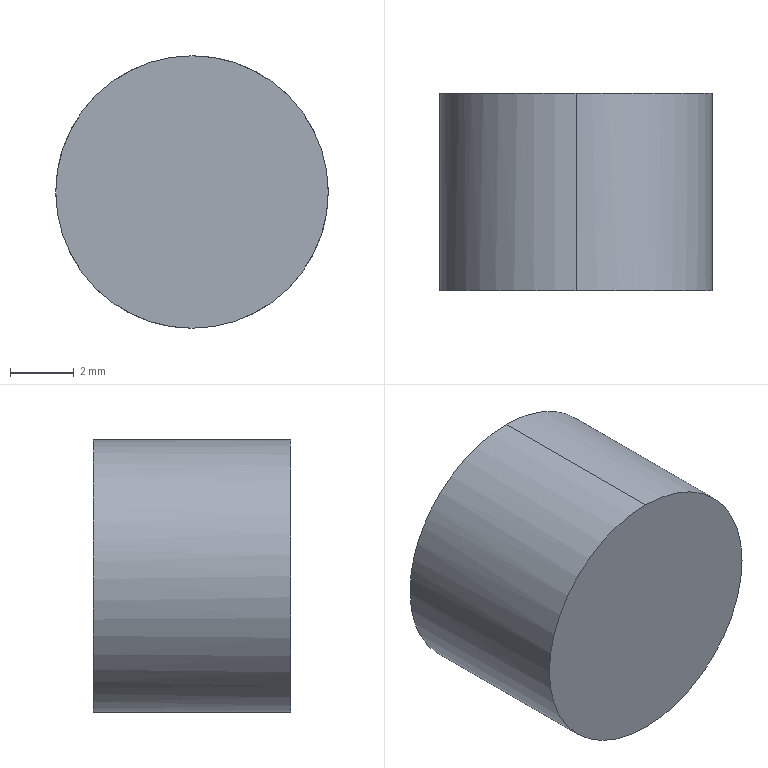Component | SolidWorks | MGPM20-20Z-M9P-1_MGP_Z_PLUG_20_9-1 | 1 solid | 11 faces | box 8.57 x 6.2 x 8.57 mm | volume 322 mm3 | plane 9 | cylinder 2 | commonest cylinder face diameters 8.566 x2
STEP:
#1=COLOUR_RGB('',0.7922,0.8196,0.9333);
#2=FILL_AREA_STYLE_COLOUR('',#1);
#3=FILL_AREA_STYLE('',(#2));
#4=SURFACE_STYLE_FILL_AREA(#3);
#5=SURFACE_SIDE_STYLE('',(#4));
#6=SURFACE_STYLE_USAGE(.BOTH.,#5);
#7=PRESENTATION_STYLE_ASSIGNMENT((#6));
#8=CARTESIAN_POINT('',(3.737,3.748,2.864));
#9=VERTEX_POINT('',#8);
#10=CARTESIAN_POINT('',(3.737,3.748,2.527));
#11=VERTEX_POINT('',#10);
#12=CARTESIAN_POINT('',(3.737,3.748,2.864));
#13=CARTESIAN_POINT('',(3.715,3.748,2.864));
#14=CARTESIAN_POINT('',(3.693,3.748,2.86));
#15=CARTESIAN_POINT('',(3.652,3.748,2.843));
#16=CARTESIAN_POINT('',(3.633,3.748,2.831));
#17=CARTESIAN_POINT('',(3.602,3.748,2.799));
#18=CARTESIAN_POINT('',(3.59,3.748,2.781));
#19=CARTESIAN_POINT('',(3.573,3.748,2.74));
#20=CARTESIAN_POINT('',(3.568,3.748,2.718));
#21=CARTESIAN_POINT('',(3.568,3.748,2.674));
#22=CARTESIAN_POINT('',(3.573,3.748,2.652));
#23=CARTESIAN_POINT('',(3.59,3.748,2.611));
#24=CARTESIAN_POINT('',(3.602,3.748,2.592));
#25=CARTESIAN_POINT('',(3.633,3.748,2.561));
#26=CARTESIAN_POINT('',(3.652,3.748,2.548));
#27=CARTESIAN_POINT('',(3.693,3.748,2.532));
#28=CARTESIAN_POINT('',(3.715,3.748,2.527));
#29=CARTESIAN_POINT('',(3.737,3.748,2.527));
#30=B_SPLINE_CURVE_WITH_KNOTS('',3,(#12,#13,#14,#15,#16,#17,#18,#19,#20,#21,#22,#23,#24,#25,#26,#27,#28,#29),.UNSPECIFIED.,.F.,.F.,(4,2,2,2,2,2,2,2,4),(0.,0.0625,0.125,0.1875,0.25,0.3125,0.375,0.4375,0.5),.UNSPECIFIED.);
#31=EDGE_CURVE('',#9,#11,#30,.T.);
#32=ORIENTED_EDGE('',*,*,#31,.T.);
#33=CARTESIAN_POINT('',(3.737,3.503,2.527));
#34=VERTEX_POINT('',#33);
#35=CARTESIAN_POINT('',(3.737,3.748,2.527));
#36=DIRECTION('',(0.,-1.,0.));
#37=VECTOR('',#36,39.37);
#38=LINE('',#35,#37);
#39=EDGE_CURVE('',#11,#34,#38,.T.);
#40=ORIENTED_EDGE('',*,*,#39,.T.);
#41=CARTESIAN_POINT('',(3.737,3.503,2.864));
#42=VERTEX_POINT('',#41);
#43=CARTESIAN_POINT('',(3.737,3.503,2.696));
#44=DIRECTION('',(0.,-1.,0.));
#45=DIRECTION('',(0.,0.,1.));
#46=AXIS2_PLACEMENT_3D('',#43,#44,#45);
#47=CIRCLE('',#46,0.1686);
#48=EDGE_CURVE('',#42,#34,#47,.T.);
#49=ORIENTED_EDGE('',*,*,#48,.F.);
#50=CARTESIAN_POINT('',(3.737,3.748,2.864));
#51=DIRECTION('',(0.,-1.,0.));
#52=VECTOR('',#51,39.37);
#53=LINE('',#50,#52);
#54=EDGE_CURVE('',#9,#42,#53,.T.);
#55=ORIENTED_EDGE('',*,*,#54,.F.);
#56=EDGE_LOOP('',(#32,#40,#49,#55));
#57=FACE_OUTER_BOUND('',#56,.T.);
#58=CARTESIAN_POINT('',(3.737,3.748,2.696));
#59=DIRECTION('',(0.,-1.,0.));
#60=DIRECTION('',(0.,0.,1.));
#61=AXIS2_PLACEMENT_3D('',#58,#59,#60);
#62=CYLINDRICAL_SURFACE('',#61,0.1686);
#63=ADVANCED_FACE('',(#57),#62,.T.);
#64=ORIENTED_EDGE('',*,*,#31,.F.);
#65=CARTESIAN_POINT('',(3.737,3.748,2.527));
#66=CARTESIAN_POINT('',(3.759,3.748,2.527));
#67=CARTESIAN_POINT('',(3.781,3.748,2.532));
#68=CARTESIAN_POINT('',(3.822,3.748,2.548));
#69=CARTESIAN_POINT('',(3.841,3.748,2.561));
#70=CARTESIAN_POINT('',(3.872,3.748,2.592));
#71=CARTESIAN_POINT('',(3.884,3.748,2.611));
#72=CARTESIAN_POINT('',(3.901,3.748,2.652));
#73=CARTESIAN_POINT('',(3.906,3.748,2.674));
#74=CARTESIAN_POINT('',(3.906,3.748,2.718));
#75=CARTESIAN_POINT('',(3.901,3.748,2.74));
#76=CARTESIAN_POINT('',(3.884,3.748,2.781));
#77=CARTESIAN_POINT('',(3.872,3.748,2.799));
#78=CARTESIAN_POINT('',(3.841,3.748,2.831));
#79=CARTESIAN_POINT('',(3.822,3.748,2.843));
#80=CARTESIAN_POINT('',(3.781,3.748,2.86));
#81=CARTESIAN_POINT('',(3.759,3.748,2.864));
#82=CARTESIAN_POINT('',(3.737,3.748,2.864));
#83=B_SPLINE_CURVE_WITH_KNOTS('',3,(#65,#66,#67,#68,#69,#70,#71,#72,#73,#74,#75,#76,#77,#78,#79,#80,#81,#82),.UNSPECIFIED.,.F.,.F.,(4,2,2,2,2,2,2,2,4),(0.5,0.5625,0.625,0.6875,0.75,0.8125,0.875,0.9375,1.),.UNSPECIFIED.);
#84=EDGE_CURVE('',#11,#9,#83,.T.);
#85=ORIENTED_EDGE('',*,*,#84,.F.);
#86=EDGE_LOOP('',(#64,#85));
#87=FACE_OUTER_BOUND('',#86,.T.);
#88=CARTESIAN_POINT('',(3.686,3.748,2.607));
#89=VERTEX_POINT('',#88);
#90=CARTESIAN_POINT('',(3.788,3.748,2.607));
#91=VERTEX_POINT('',#90);
#92=CARTESIAN_POINT('',(3.686,3.748,2.607));
#93=DIRECTION('',(1.,0.,-0.));
#94=VECTOR('',#93,39.37);
#95=LINE('',#92,#94);
#96=EDGE_CURVE('',#89,#91,#95,.T.);
#97=ORIENTED_EDGE('',*,*,#96,.T.);
#98=CARTESIAN_POINT('',(3.839,3.748,2.696));
#99=VERTEX_POINT('',#98);
#100=CARTESIAN_POINT('',(3.788,3.748,2.607));
#101=DIRECTION('',(0.5,0.,0.866));
#102=VECTOR('',#101,39.37);
#103=LINE('',#100,#102);
#104=EDGE_CURVE('',#91,#99,#103,.T.);
#105=ORIENTED_EDGE('',*,*,#104,.T.);
#106=CARTESIAN_POINT('',(3.788,3.748,2.784));
#107=VERTEX_POINT('',#106);
#108=CARTESIAN_POINT('',(3.839,3.748,2.696));
#109=DIRECTION('',(-0.5,0.,0.866));
#110=VECTOR('',#109,39.37);
#111=LINE('',#108,#110);
#112=EDGE_CURVE('',#99,#107,#111,.T.);
#113=ORIENTED_EDGE('',*,*,#112,.T.);
#114=CARTESIAN_POINT('',(3.686,3.748,2.784));
#115=VERTEX_POINT('',#114);
#116=CARTESIAN_POINT('',(3.788,3.748,2.784));
#117=DIRECTION('',(-1.,-0.,0.));
#118=VECTOR('',#117,39.37);
#119=LINE('',#116,#118);
#120=EDGE_CURVE('',#107,#115,#119,.T.);
#121=ORIENTED_EDGE('',*,*,#120,.T.);
#122=CARTESIAN_POINT('',(3.635,3.748,2.696));
#123=VERTEX_POINT('',#122);
#124=CARTESIAN_POINT('',(3.686,3.748,2.784));
#125=DIRECTION('',(-0.5,-0.,-0.866));
#126=VECTOR('',#125,39.37);
#127=LINE('',#124,#126);
#128=EDGE_CURVE('',#115,#123,#127,.T.);
#129=ORIENTED_EDGE('',*,*,#128,.T.);
#130=CARTESIAN_POINT('',(3.635,3.748,2.696));
#131=DIRECTION('',(0.5,-0.,-0.866));
#132=VECTOR('',#131,39.37);
#133=LINE('',#130,#132);
#134=EDGE_CURVE('',#123,#89,#133,.T.);
#135=ORIENTED_EDGE('',*,*,#134,.T.);
#136=EDGE_LOOP('',(#97,#105,#113,#121,#129,#135));
#137=FACE_BOUND('',#136,.T.);
#138=CARTESIAN_POINT('',(3.737,3.748,2.696));
#139=DIRECTION('',(0.,-1.,0.));
#140=DIRECTION('',(0.,0.,1.));
#141=AXIS2_PLACEMENT_3D('',#138,#139,#140);
#142=PLANE('',#141);
#143=ADVANCED_FACE('',(#87,#137),#142,.F.);
#144=ORIENTED_EDGE('',*,*,#134,.F.);
#145=CARTESIAN_POINT('',(3.635,3.669,2.696));
#146=VERTEX_POINT('',#145);
#147=CARTESIAN_POINT('',(3.635,3.669,2.696));
#148=DIRECTION('',(-0.,1.,-0.));
#149=VECTOR('',#148,39.37);
#150=LINE('',#147,#149);
#151=EDGE_CURVE('',#146,#123,#150,.T.);
#152=ORIENTED_EDGE('',*,*,#151,.F.);
#153=CARTESIAN_POINT('',(3.686,3.669,2.607));
#154=VERTEX_POINT('',#153);
#155=CARTESIAN_POINT('',(3.635,3.669,2.696));
#156=DIRECTION('',(0.5,-0.,-0.866));
#157=VECTOR('',#156,39.37);
#158=LINE('',#155,#157);
#159=EDGE_CURVE('',#146,#154,#158,.T.);
#160=ORIENTED_EDGE('',*,*,#159,.T.);
#161=CARTESIAN_POINT('',(3.686,3.669,2.607));
#162=DIRECTION('',(-0.,1.,-0.));
#163=VECTOR('',#162,39.37);
#164=LINE('',#161,#163);
#165=EDGE_CURVE('',#154,#89,#164,.T.);
#166=ORIENTED_EDGE('',*,*,#165,.T.);
#167=EDGE_LOOP('',(#144,#152,#160,#166));
#168=FACE_OUTER_BOUND('',#167,.T.);
#169=CARTESIAN_POINT('',(3.635,3.669,2.696));
#170=DIRECTION('',(0.866,0.,0.5));
#171=DIRECTION('',(-0.5,0.,0.866));
#172=AXIS2_PLACEMENT_3D('',#169,#170,#171);
#173=PLANE('',#172);
#174=ADVANCED_FACE('',(#168),#173,.T.);
#175=ORIENTED_EDGE('',*,*,#96,.F.);
#176=ORIENTED_EDGE('',*,*,#165,.F.);
#177=CARTESIAN_POINT('',(3.788,3.669,2.607));
#178=VERTEX_POINT('',#177);
#179=CARTESIAN_POINT('',(3.686,3.669,2.607));
#180=DIRECTION('',(1.,0.,-0.));
#181=VECTOR('',#180,39.37);
#182=LINE('',#179,#181);
#183=EDGE_CURVE('',#154,#178,#182,.T.);
#184=ORIENTED_EDGE('',*,*,#183,.T.);
#185=CARTESIAN_POINT('',(3.788,3.669,2.607));
#186=DIRECTION('',(-0.,1.,-0.));
#187=VECTOR('',#186,39.37);
#188=LINE('',#185,#187);
#189=EDGE_CURVE('',#178,#91,#188,.T.);
#190=ORIENTED_EDGE('',*,*,#189,.T.);
#191=EDGE_LOOP('',(#175,#176,#184,#190));
#192=FACE_OUTER_BOUND('',#191,.T.);
#193=CARTESIAN_POINT('',(3.686,3.669,2.607));
#194=DIRECTION('',(0.,0.,1.));
#195=DIRECTION('',(-0.,1.,-0.));
#196=AXIS2_PLACEMENT_3D('',#193,#194,#195);
#197=PLANE('',#196);
#198=ADVANCED_FACE('',(#192),#197,.T.);
#199=ORIENTED_EDGE('',*,*,#104,.F.);
#200=ORIENTED_EDGE('',*,*,#189,.F.);
#201=CARTESIAN_POINT('',(3.839,3.669,2.696));
#202=VERTEX_POINT('',#201);
#203=CARTESIAN_POINT('',(3.788,3.669,2.607));
#204=DIRECTION('',(0.5,0.,0.866));
#205=VECTOR('',#204,39.37);
#206=LINE('',#203,#205);
#207=EDGE_CURVE('',#178,#202,#206,.T.);
#208=ORIENTED_EDGE('',*,*,#207,.T.);
#209=CARTESIAN_POINT('',(3.839,3.669,2.696));
#210=DIRECTION('',(-0.,1.,-0.));
#211=VECTOR('',#210,39.37);
#212=LINE('',#209,#211);
#213=EDGE_CURVE('',#202,#99,#212,.T.);
#214=ORIENTED_EDGE('',*,*,#213,.T.);
#215=EDGE_LOOP('',(#199,#200,#208,#214));
#216=FACE_OUTER_BOUND('',#215,.T.);
#217=CARTESIAN_POINT('',(3.788,3.669,2.607));
#218=DIRECTION('',(-0.866,0.,0.5));
#219=DIRECTION('',(-0.5,-0.,-0.866));
#220=AXIS2_PLACEMENT_3D('',#217,#218,#219);
#221=PLANE('',#220);
#222=ADVANCED_FACE('',(#216),#221,.T.);
#223=ORIENTED_EDGE('',*,*,#112,.F.);
#224=ORIENTED_EDGE('',*,*,#213,.F.);
#225=CARTESIAN_POINT('',(3.788,3.669,2.784));
#226=VERTEX_POINT('',#225);
#227=CARTESIAN_POINT('',(3.839,3.669,2.696));
#228=DIRECTION('',(-0.5,0.,0.866));
#229=VECTOR('',#228,39.37);
#230=LINE('',#227,#229);
#231=EDGE_CURVE('',#202,#226,#230,.T.);
#232=ORIENTED_EDGE('',*,*,#231,.T.);
#233=CARTESIAN_POINT('',(3.788,3.669,2.784));
#234=DIRECTION('',(-0.,1.,-0.));
#235=VECTOR('',#234,39.37);
#236=LINE('',#233,#235);
#237=EDGE_CURVE('',#226,#107,#236,.T.);
#238=ORIENTED_EDGE('',*,*,#237,.T.);
#239=EDGE_LOOP('',(#223,#224,#232,#238));
#240=FACE_OUTER_BOUND('',#239,.T.);
#241=CARTESIAN_POINT('',(3.839,3.669,2.696));
#242=DIRECTION('',(-0.866,-0.,-0.5));
#243=DIRECTION('',(0.5,-0.,-0.866));
#244=AXIS2_PLACEMENT_3D('',#241,#242,#243);
#245=PLANE('',#244);
#246=ADVANCED_FACE('',(#240),#245,.T.);
#247=ORIENTED_EDGE('',*,*,#120,.F.);
#248=ORIENTED_EDGE('',*,*,#237,.F.);
#249=CARTESIAN_POINT('',(3.686,3.669,2.784));
#250=VERTEX_POINT('',#249);
#251=CARTESIAN_POINT('',(3.788,3.669,2.784));
#252=DIRECTION('',(-1.,-0.,0.));
#253=VECTOR('',#252,39.37);
#254=LINE('',#251,#253);
#255=EDGE_CURVE('',#226,#250,#254,.T.);
#256=ORIENTED_EDGE('',*,*,#255,.T.);
#257=CARTESIAN_POINT('',(3.686,3.669,2.784));
#258=DIRECTION('',(-0.,1.,-0.));
#259=VECTOR('',#258,39.37);
#260=LINE('',#257,#259);
#261=EDGE_CURVE('',#250,#115,#260,.T.);
#262=ORIENTED_EDGE('',*,*,#261,.T.);
#263=EDGE_LOOP('',(#247,#248,#256,#262));
#264=FACE_OUTER_BOUND('',#263,.T.);
#265=CARTESIAN_POINT('',(3.788,3.669,2.784));
#266=DIRECTION('',(-0.,-0.,-1.));
#267=DIRECTION('',(0.,-1.,0.));
#268=AXIS2_PLACEMENT_3D('',#265,#266,#267);
#269=PLANE('',#268);
#270=ADVANCED_FACE('',(#264),#269,.T.);
#271=ORIENTED_EDGE('',*,*,#128,.F.);
#272=ORIENTED_EDGE('',*,*,#261,.F.);
#273=CARTESIAN_POINT('',(3.686,3.669,2.784));
#274=DIRECTION('',(-0.5,-0.,-0.866));
#275=VECTOR('',#274,39.37);
#276=LINE('',#273,#275);
#277=EDGE_CURVE('',#250,#146,#276,.T.);
#278=ORIENTED_EDGE('',*,*,#277,.T.);
#279=ORIENTED_EDGE('',*,*,#151,.T.);
#280=EDGE_LOOP('',(#271,#272,#278,#279));
#281=FACE_OUTER_BOUND('',#280,.T.);
#282=CARTESIAN_POINT('',(3.686,3.669,2.784));
#283=DIRECTION('',(0.866,-0.,-0.5));
#284=DIRECTION('',(0.5,0.,0.866));
#285=AXIS2_PLACEMENT_3D('',#282,#283,#284);
#286=PLANE('',#285);
#287=ADVANCED_FACE('',(#281),#286,.T.);
#288=ORIENTED_EDGE('',*,*,#183,.F.);
#289=ORIENTED_EDGE('',*,*,#159,.F.);
#290=ORIENTED_EDGE('',*,*,#277,.F.);
#291=ORIENTED_EDGE('',*,*,#255,.F.);
#292=ORIENTED_EDGE('',*,*,#231,.F.);
#293=ORIENTED_EDGE('',*,*,#207,.F.);
#294=EDGE_LOOP('',(#288,#289,#290,#291,#292,#293));
#295=FACE_OUTER_BOUND('',#294,.T.);
#296=CARTESIAN_POINT('',(3.737,3.669,2.696));
#297=DIRECTION('',(0.,-1.,0.));
#298=DIRECTION('',(0.,0.,1.));
#299=AXIS2_PLACEMENT_3D('',#296,#297,#298);
#300=PLANE('',#299);
#301=ADVANCED_FACE('',(#295),#300,.F.);
#302=ORIENTED_EDGE('',*,*,#39,.F.);
#303=ORIENTED_EDGE('',*,*,#84,.T.);
#304=ORIENTED_EDGE('',*,*,#54,.T.);
#305=CARTESIAN_POINT('',(3.737,3.503,2.696));
#306=DIRECTION('',(0.,-1.,0.));
#307=DIRECTION('',(0.,0.,1.));
#308=AXIS2_PLACEMENT_3D('',#305,#306,#307);
#309=CIRCLE('',#308,0.1686);
#310=EDGE_CURVE('',#34,#42,#309,.T.);
#311=ORIENTED_EDGE('',*,*,#310,.F.);
#312=EDGE_LOOP('',(#302,#303,#304,#311));
#313=FACE_OUTER_BOUND('',#312,.T.);
#314=CARTESIAN_POINT('',(3.737,3.748,2.696));
#315=DIRECTION('',(0.,-1.,0.));
#316=DIRECTION('',(0.,0.,1.));
#317=AXIS2_PLACEMENT_3D('',#314,#315,#316);
#318=CYLINDRICAL_SURFACE('',#317,0.1686);
#319=ADVANCED_FACE('',(#313),#318,.T.);
#320=ORIENTED_EDGE('',*,*,#48,.T.);
#321=ORIENTED_EDGE('',*,*,#310,.T.);
#322=EDGE_LOOP('',(#320,#321));
#323=FACE_OUTER_BOUND('',#322,.T.);
#324=CARTESIAN_POINT('',(3.568,3.503,2.696));
#325=DIRECTION('',(-0.,1.,-0.));
#326=DIRECTION('',(-0.,-0.,-1.));
#327=AXIS2_PLACEMENT_3D('',#324,#325,#326);
#328=PLANE('',#327);
#329=ADVANCED_FACE('',(#323),#328,.F.);
#330=CLOSED_SHELL('',(#63,#143,#174,#198,#222,#246,#270,#287,#301,#319,#329));
#331=MANIFOLD_SOLID_BREP('',#330);
#332=STYLED_ITEM('',(#7),#331);
#333=PRESENTATION_LAYER_ASSIGNMENT('','',(#332));
#334=CARTESIAN_POINT('',(0.,0.,0.));
#335=DIRECTION('',(0.,0.,1.));
#336=DIRECTION('',(1.,0.,0.));
#337=AXIS2_PLACEMENT_3D('',#334,#335,#336);
#338=(LENGTH_UNIT()NAMED_UNIT(*)SI_UNIT($,.METRE.));
#339=LENGTH_MEASURE_WITH_UNIT(LENGTH_MEASURE(0.0254),#338);
#340=DIMENSIONAL_EXPONENTS(1.,0.,0.,0.,0.,0.,0.);
#341=(CONVERSION_BASED_UNIT('',#339)LENGTH_UNIT()NAMED_UNIT(#340));
#342=UNCERTAINTY_MEASURE_WITH_UNIT(LENGTH_MEASURE(0.00001),#341,'','');
#343=(NAMED_UNIT(*)PLANE_ANGLE_UNIT()SI_UNIT($,.RADIAN.));
#344=(NAMED_UNIT(*)SI_UNIT($,.STERADIAN.)SOLID_ANGLE_UNIT());
#345=(GEOMETRIC_REPRESENTATION_CONTEXT(3)GLOBAL_UNCERTAINTY_ASSIGNED_CONTEXT((#342))GLOBAL_UNIT_ASSIGNED_CONTEXT((#341,#343,#344))REPRESENTATION_CONTEXT('',''));
#346=ADVANCED_BREP_SHAPE_REPRESENTATION('',(#331,#337),#345);
#347=(LENGTH_UNIT()NAMED_UNIT(*)SI_UNIT($,.METRE.));
#348=LENGTH_MEASURE_WITH_UNIT(LENGTH_MEASURE(0.0254),#347);
#349=DIMENSIONAL_EXPONENTS(1.,0.,0.,0.,0.,0.,0.);
#350=(CONVERSION_BASED_UNIT('',#348)LENGTH_UNIT()NAMED_UNIT(#349));
#351=UNCERTAINTY_MEASURE_WITH_UNIT(LENGTH_MEASURE(0.00001),#350,'','');
#352=(NAMED_UNIT(*)PLANE_ANGLE_UNIT()SI_UNIT($,.RADIAN.));
#353=(NAMED_UNIT(*)SI_UNIT($,.STERADIAN.)SOLID_ANGLE_UNIT());
#354=(GEOMETRIC_REPRESENTATION_CONTEXT(3)GLOBAL_UNCERTAINTY_ASSIGNED_CONTEXT((#351))GLOBAL_UNIT_ASSIGNED_CONTEXT((#350,#352,#353))REPRESENTATION_CONTEXT('',''));
#355=MECHANICAL_DESIGN_GEOMETRIC_PRESENTATION_REPRESENTATION('',(#332),#354);